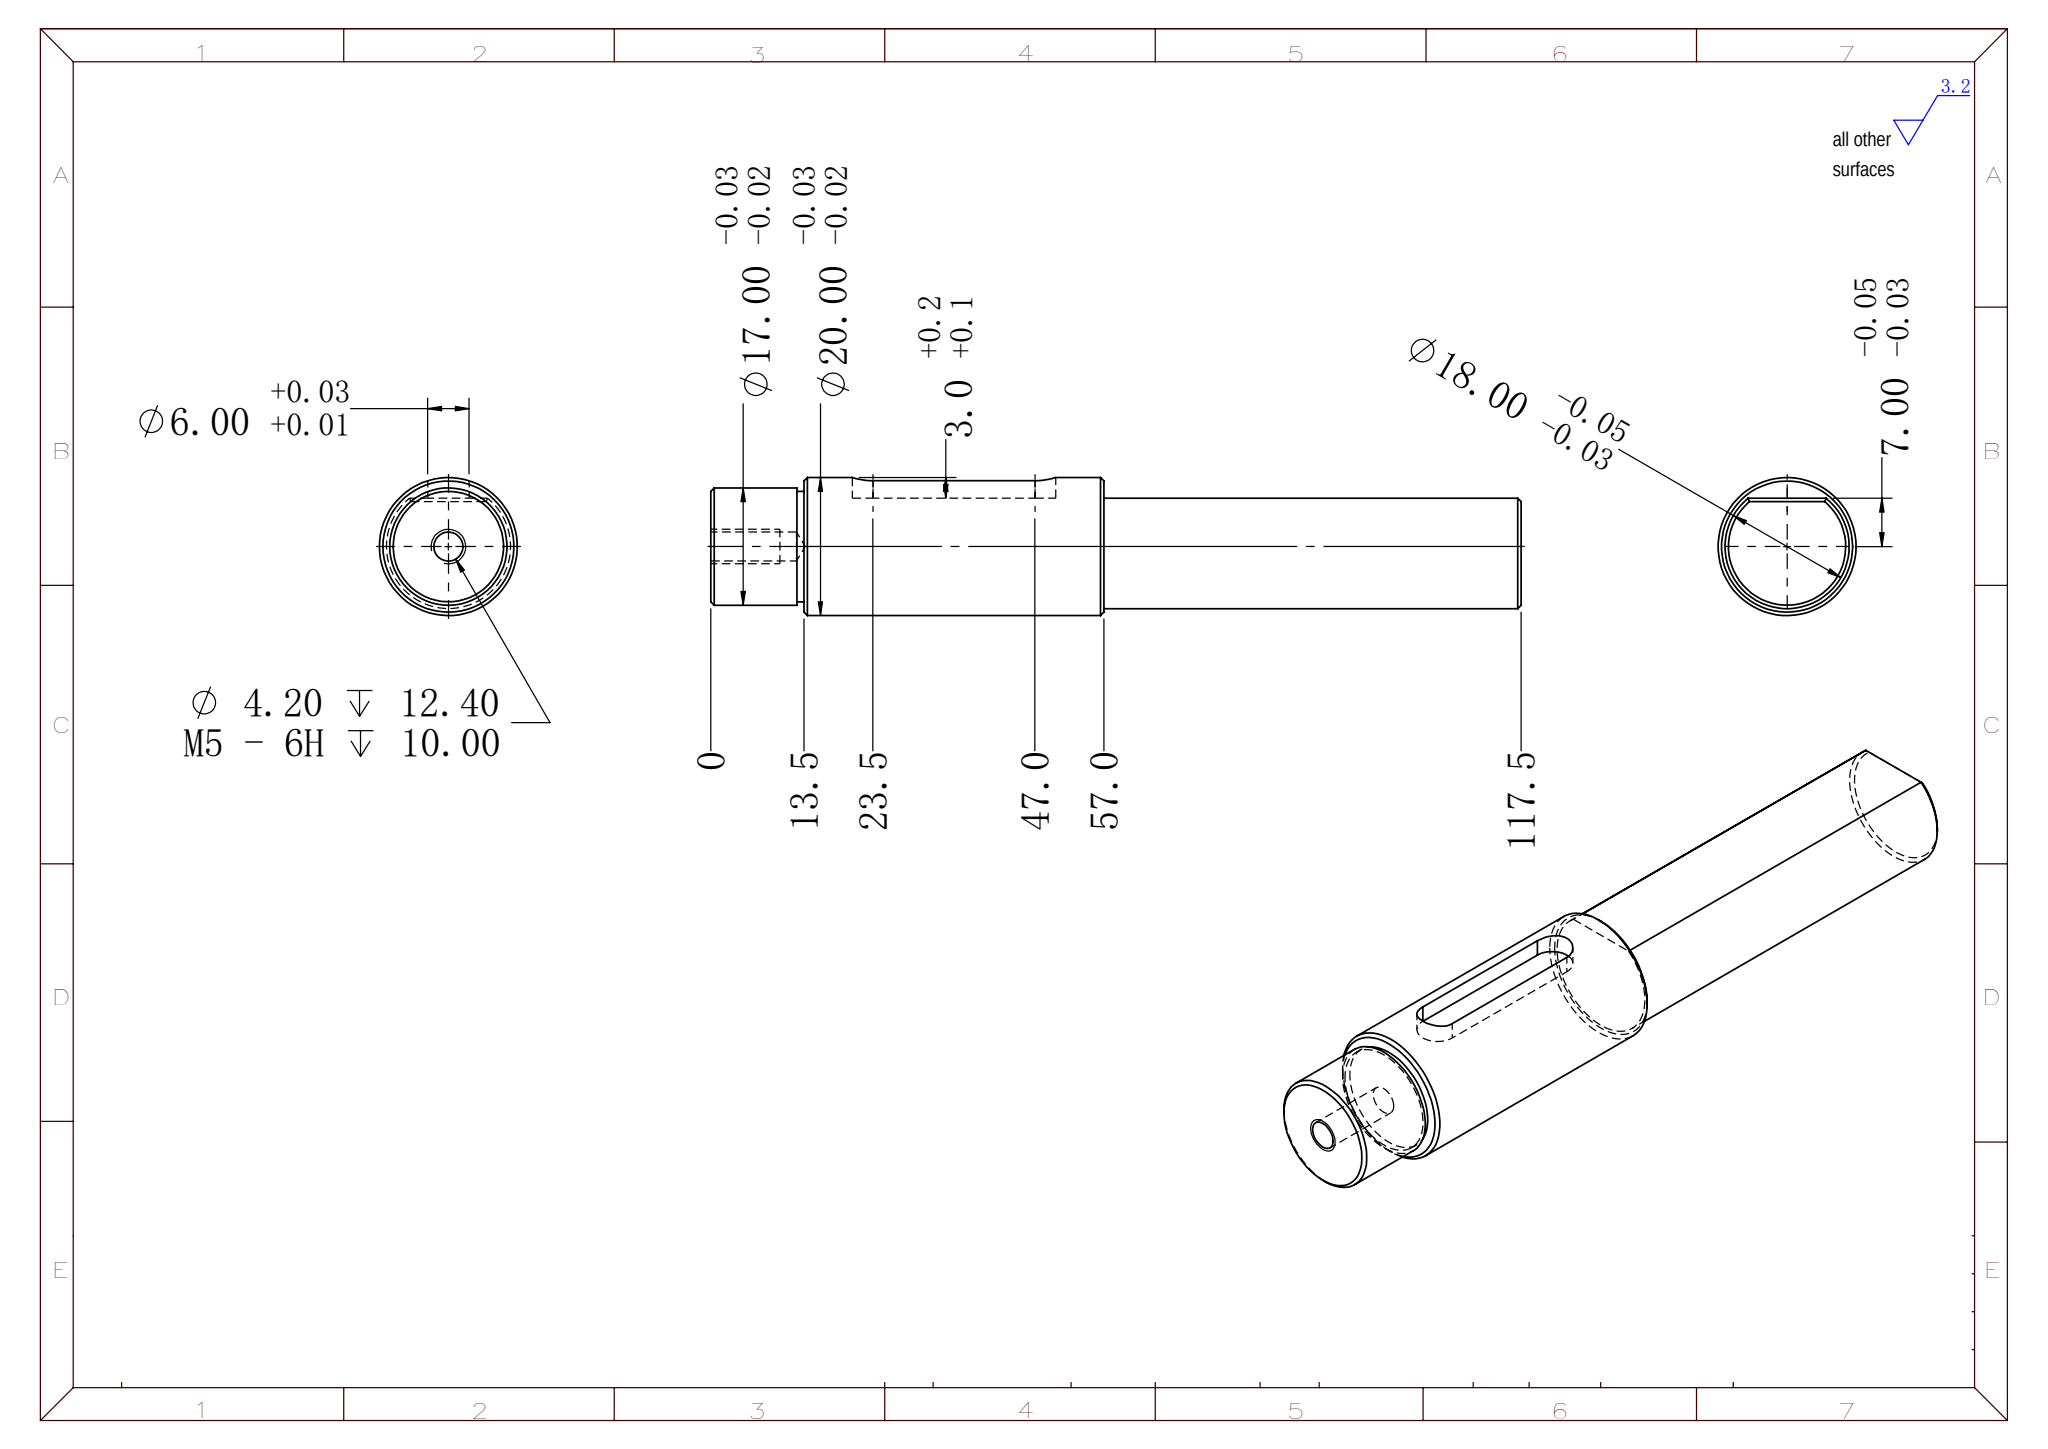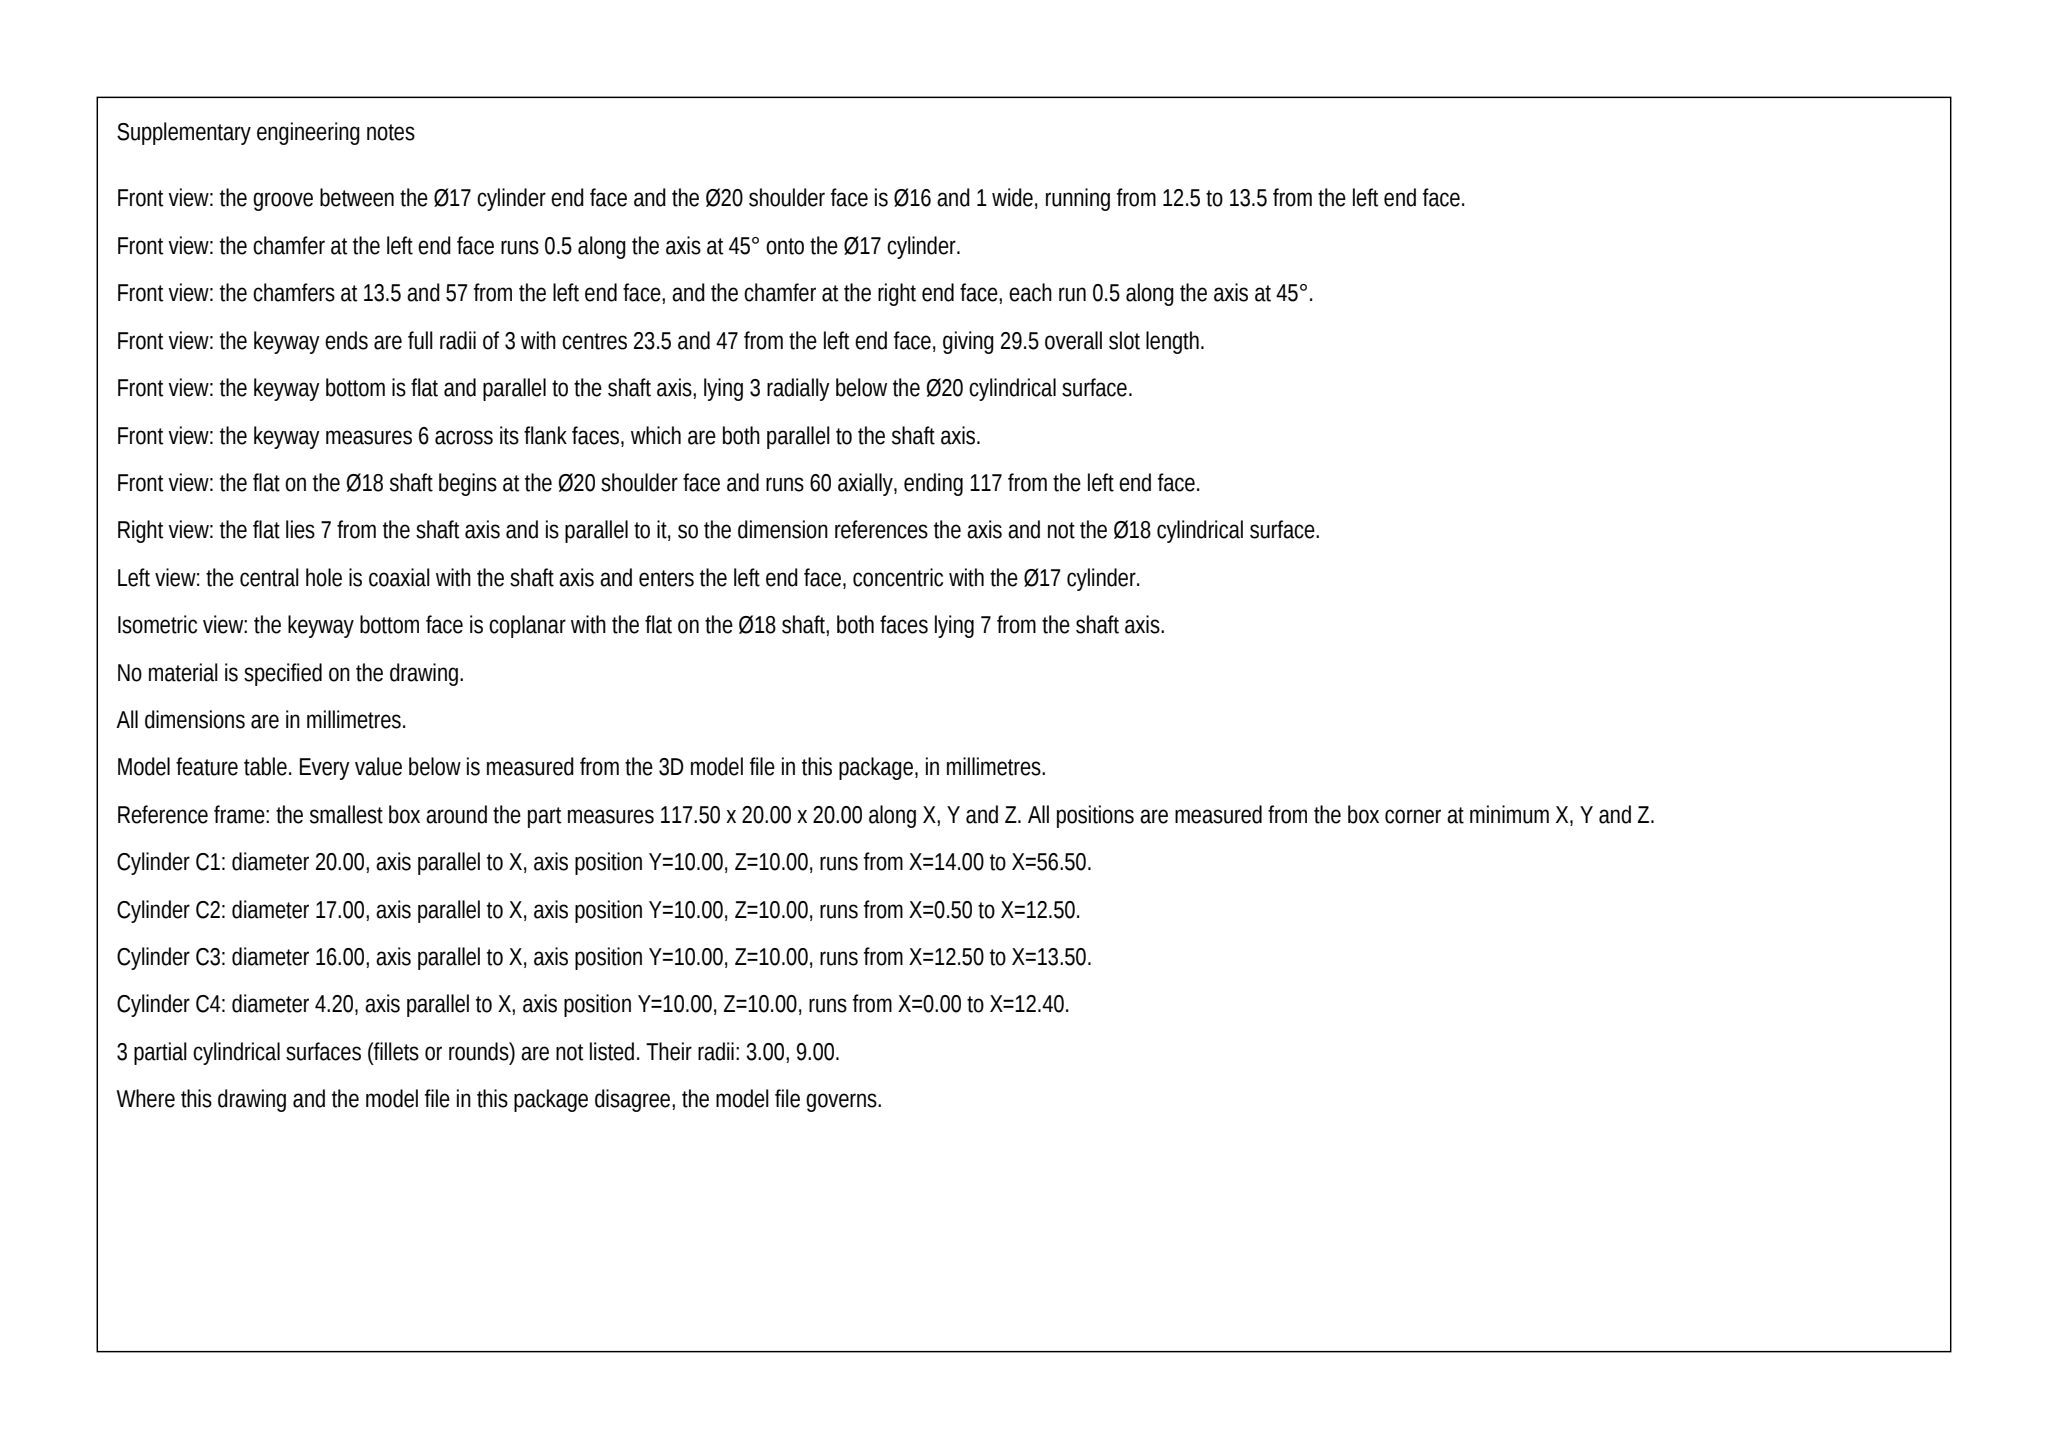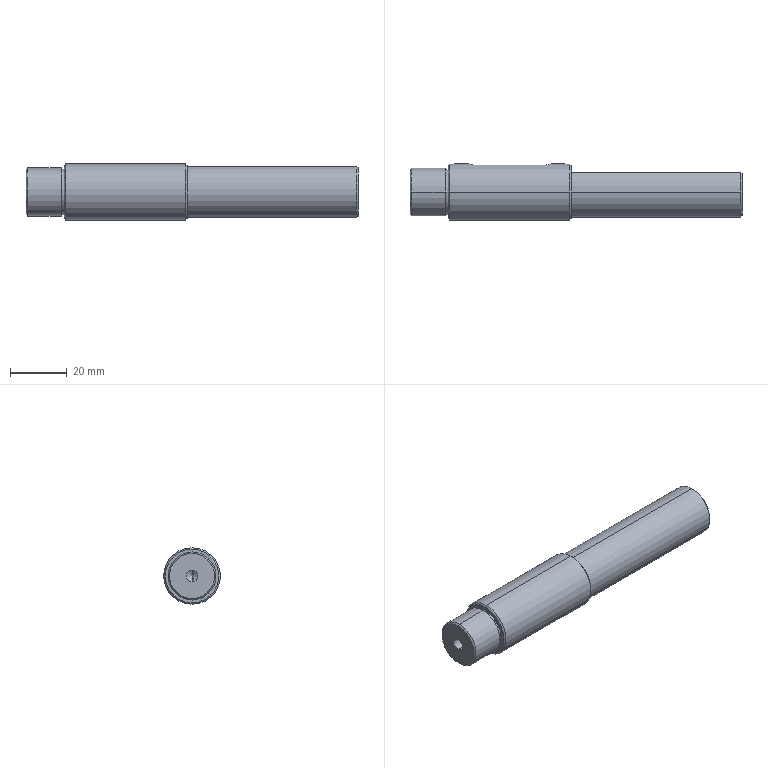Part | SolidWorks | mm | 1 solid | 34 faces | box 117.5 x 20 x 20 mm | volume 30475 mm3 | cylinder 13 | cone 11 | plane 10 | commonest cylinder face diameters 18 x3 4.2 x2 16 x2 17 x2 20 x2 6 x2
Drawing notes:
GROOVE Ø16 x 1.0 WIDE, 12.5 TO 13.5 FROM Ø17 END FACE | from the solid: Ø16 cyl, axis x, L=1.0; x-planes at 12.5 and 13.5; Ø17 step 0-12.5 from x=0 end face
ALL CHAMFERS 45°: C1 AT Ø20-Ø18 STEP, C0.5 ELSEWHERE | from the solid: cones all 90° incl ang (=45°); ref_dia 19 cone between Ø20 (ends x=56.0) and Ø18 (starts x=57.0) = 1.0 leg; Ø17 cyl L=12 within 0-12.5 = 0.5 leg
FLAT ON Ø18: 7.00 FROM AXIS, 57.0 TO 117.5 FROM Ø17 END | from the solid: y-plane offset 17.0 (axis y=10.0 -> 7.00); Ø18 shank x=57.0 to bbox end 117.5
FLAT ON Ø18 (7.00 FROM AXIS) SAME SIDE AS Ø6 SLOT, 0 DEG APART | from the solid: Flat plane y=17.0 and keyway bottom plane y=17.0 share same normal/offset; axis at y=10, so both features lie on +Y side, 7.00 from axis